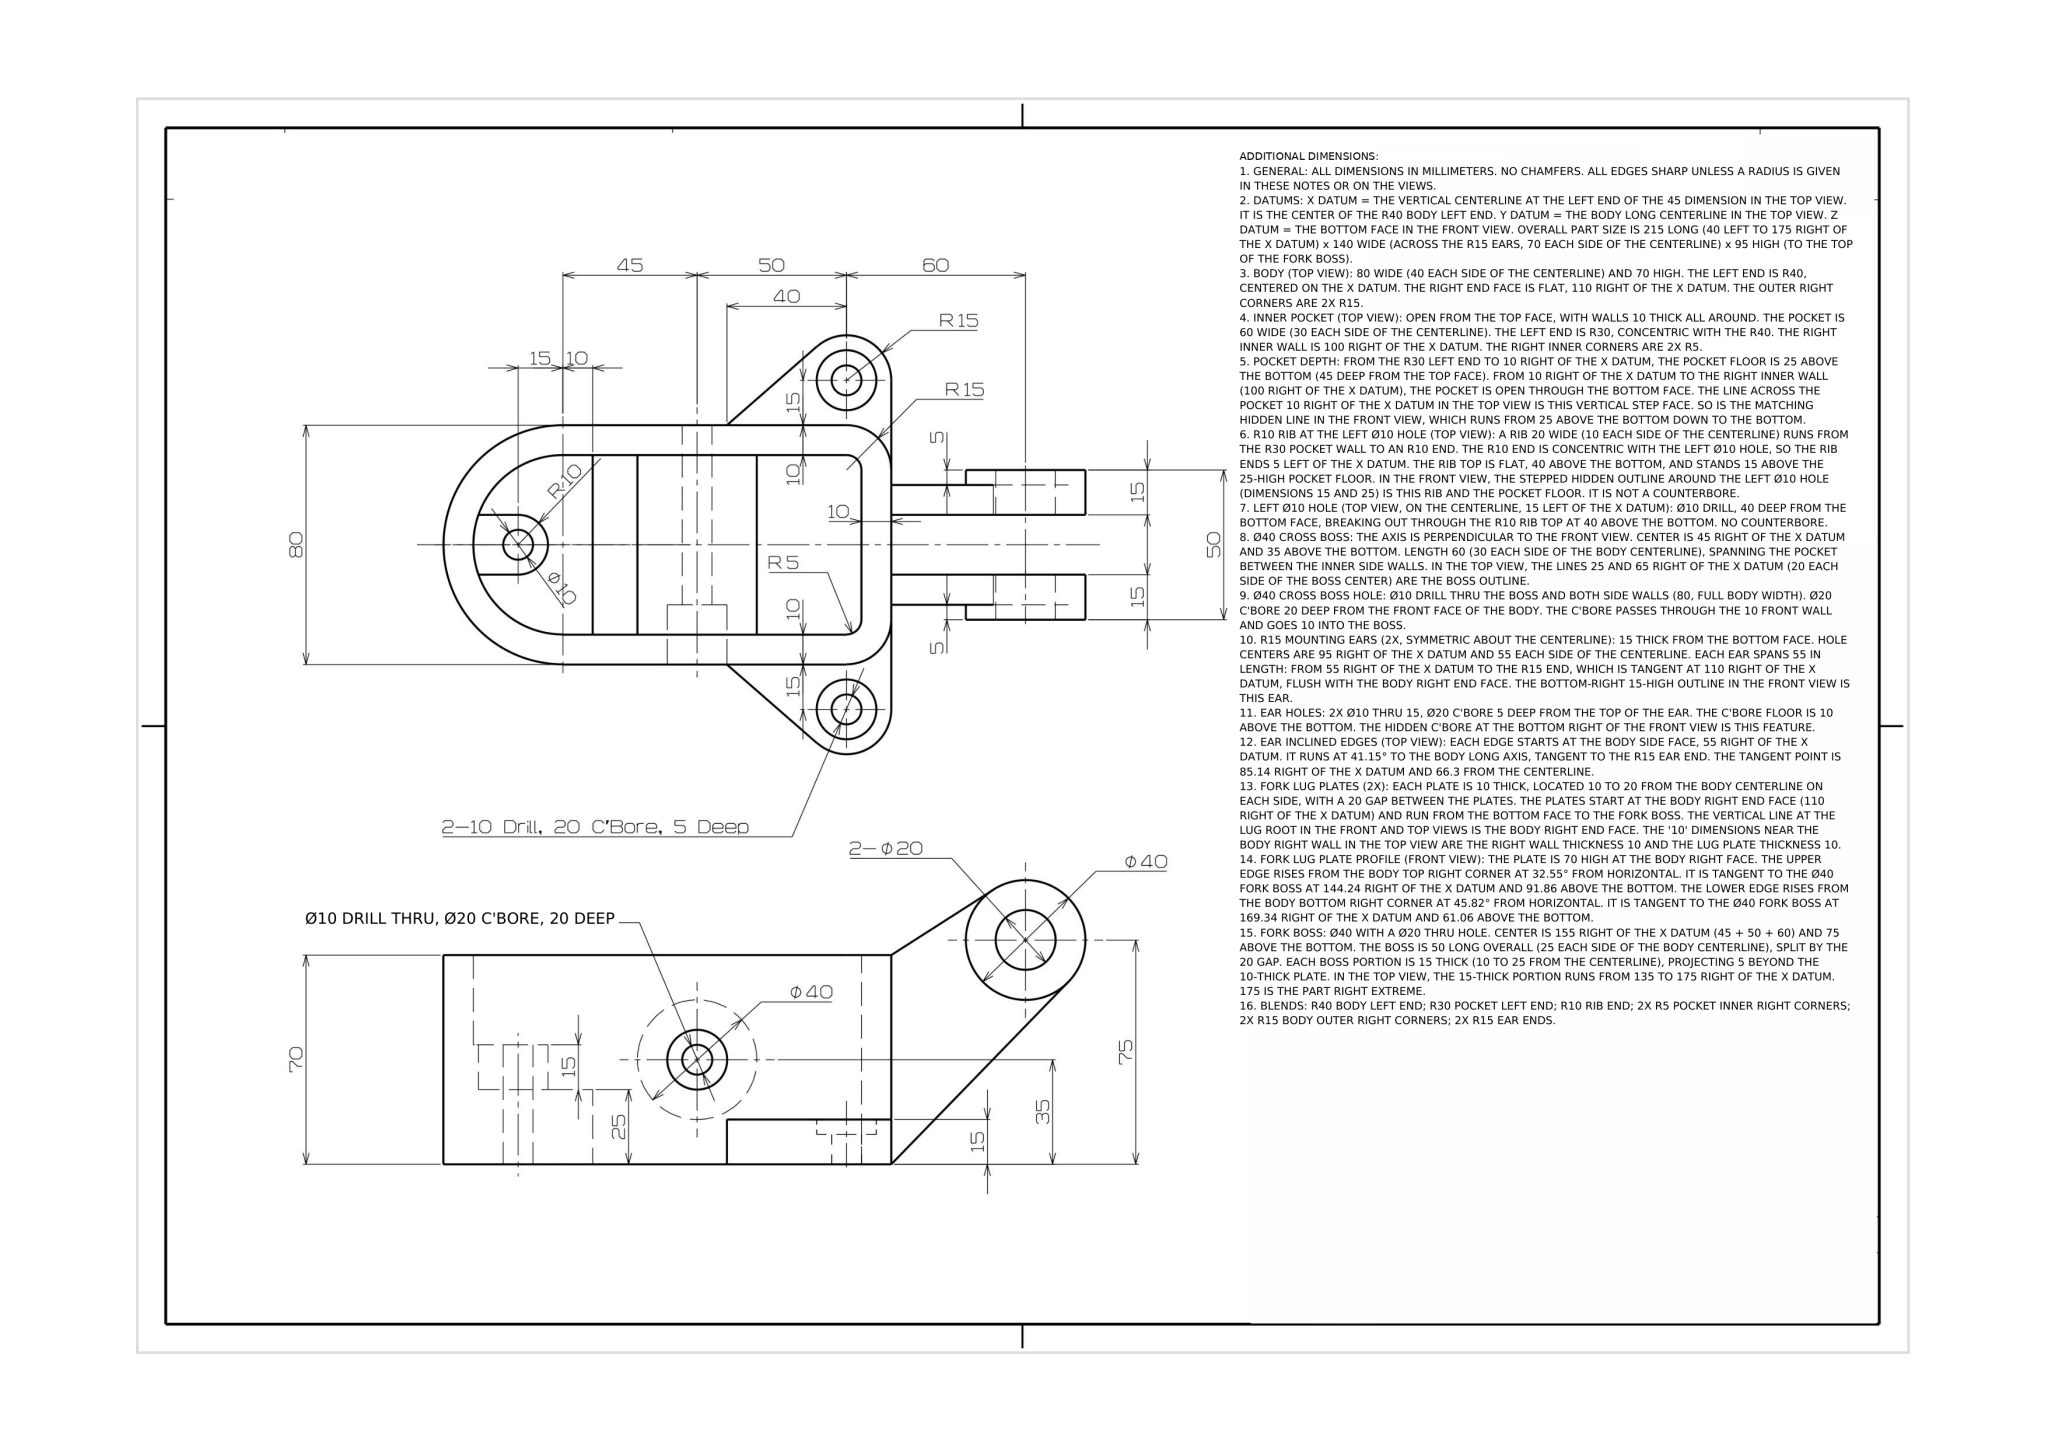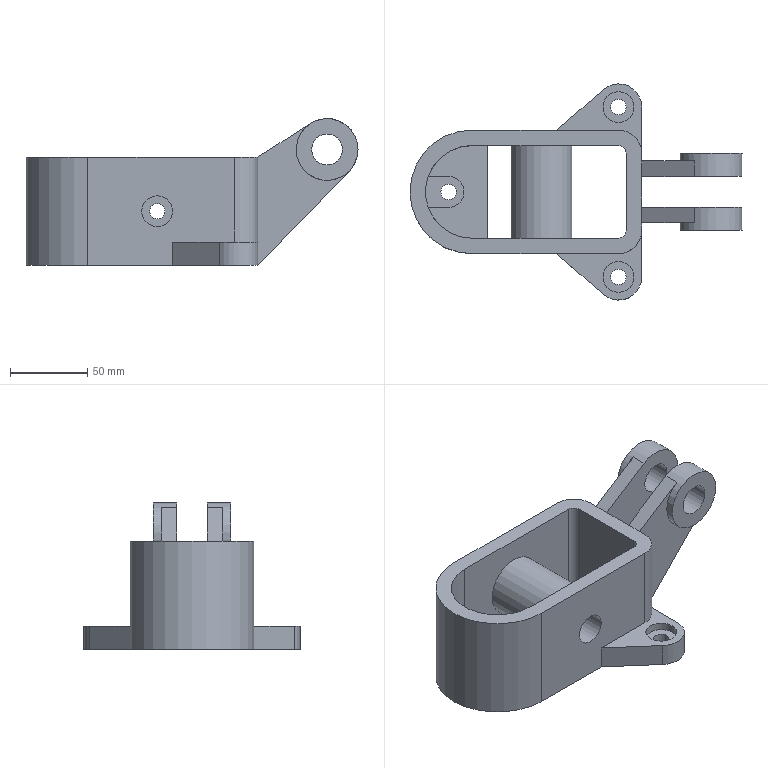Part | NX | mm | 1 solid | 53 faces | box 215 x 140 x 95 mm | volume 485896 mm3 | plane 32 | cylinder 21 | commonest cylinder face diameters 10 x6 20 x6 30 x4 40 x3 80 x1 60 x1